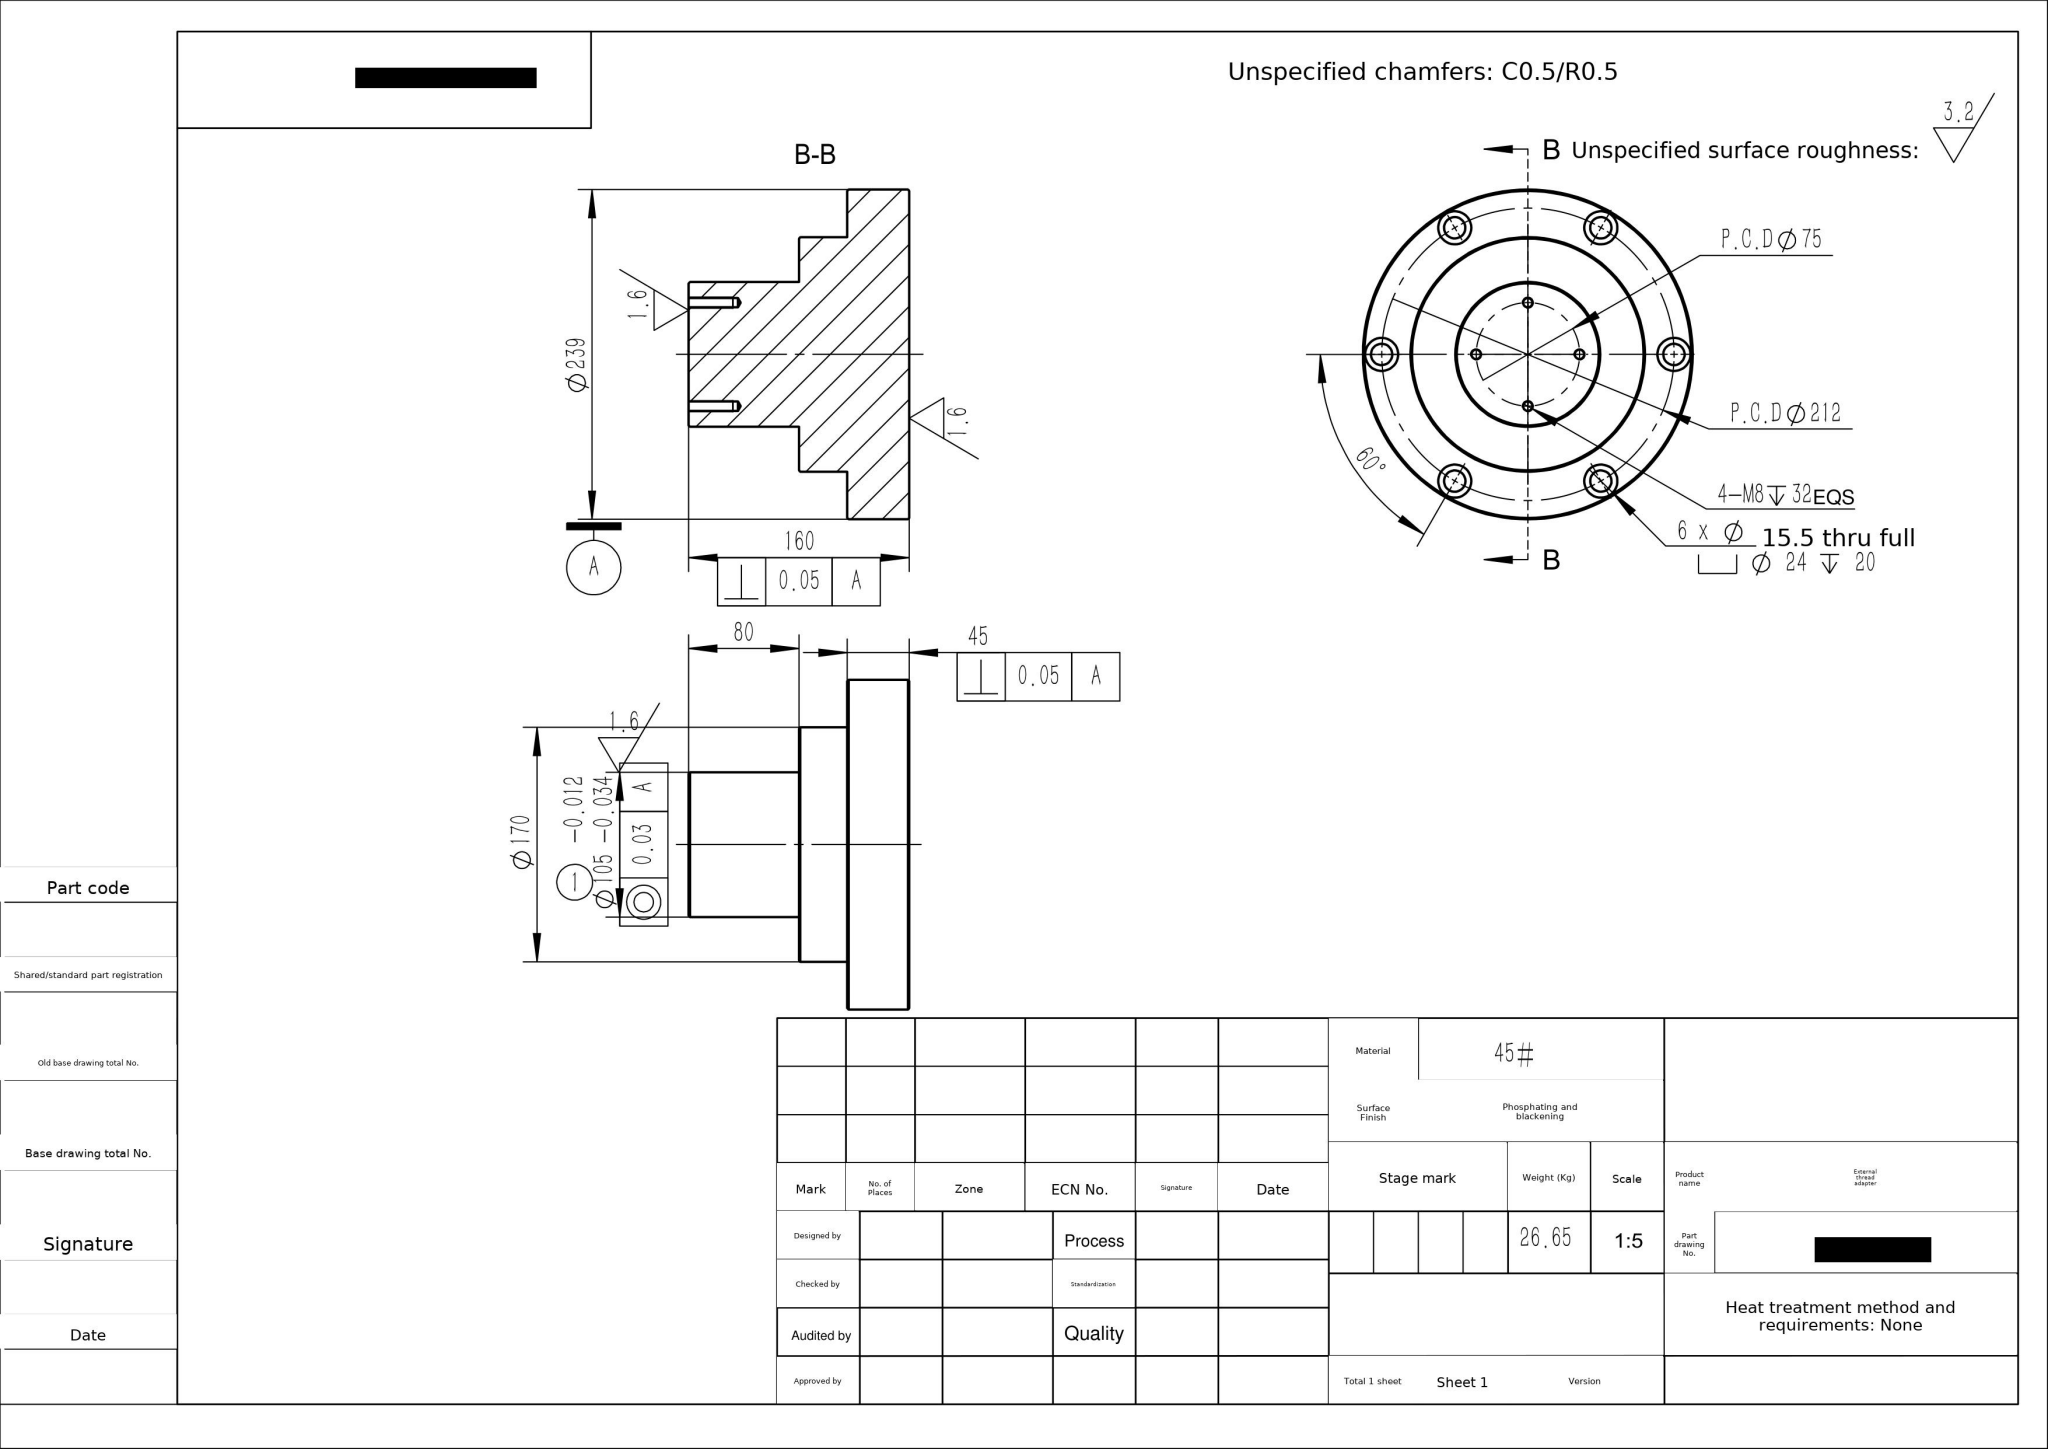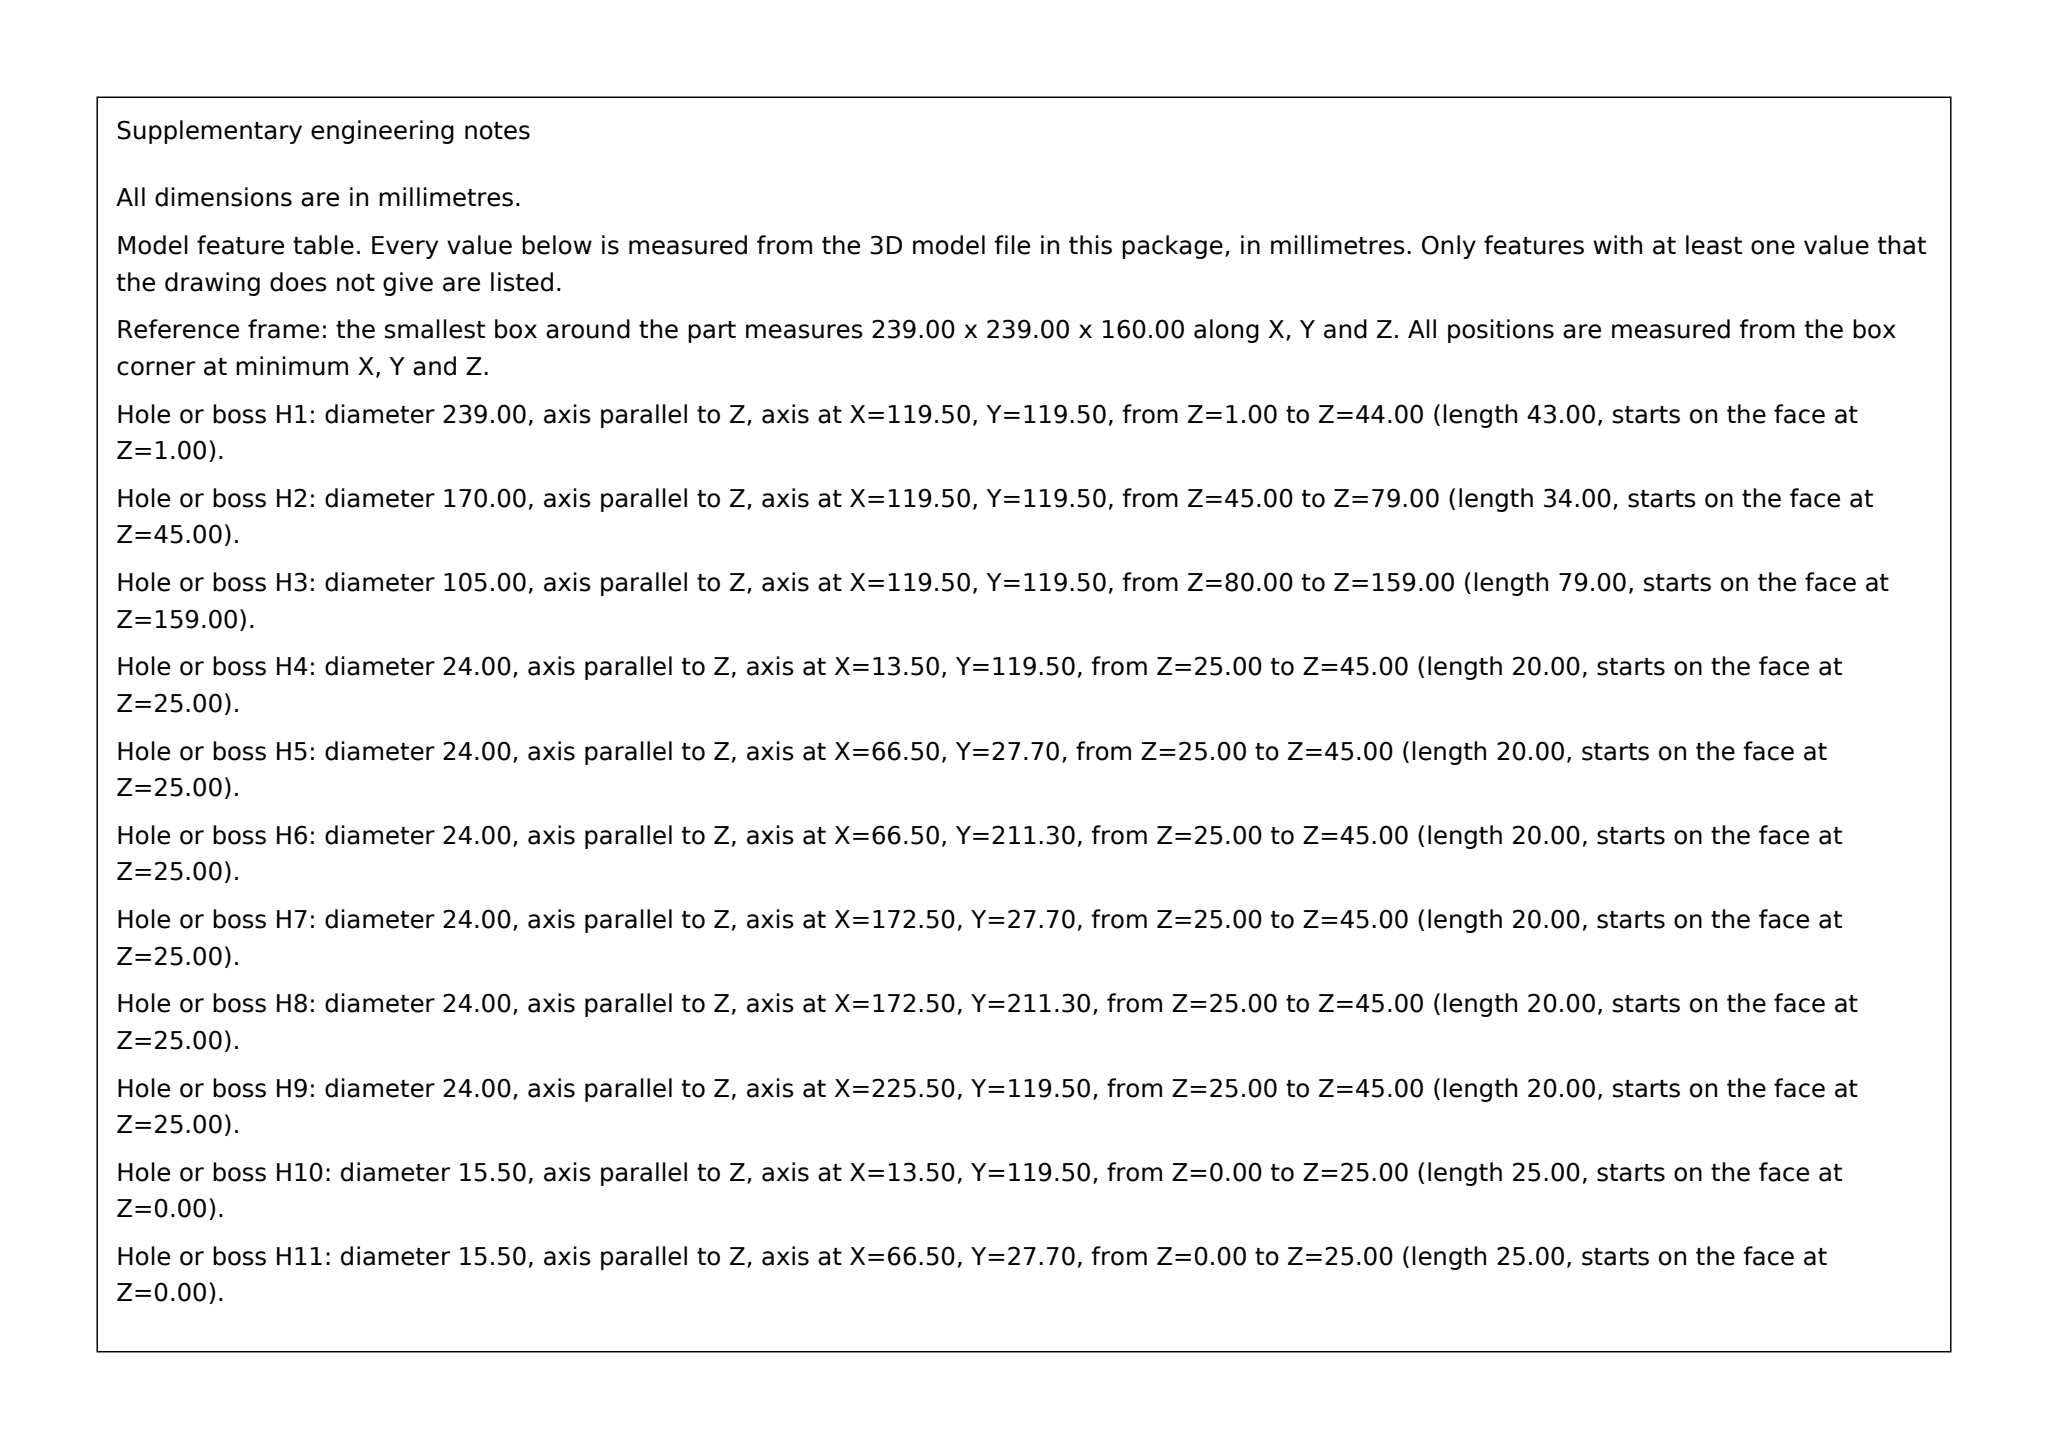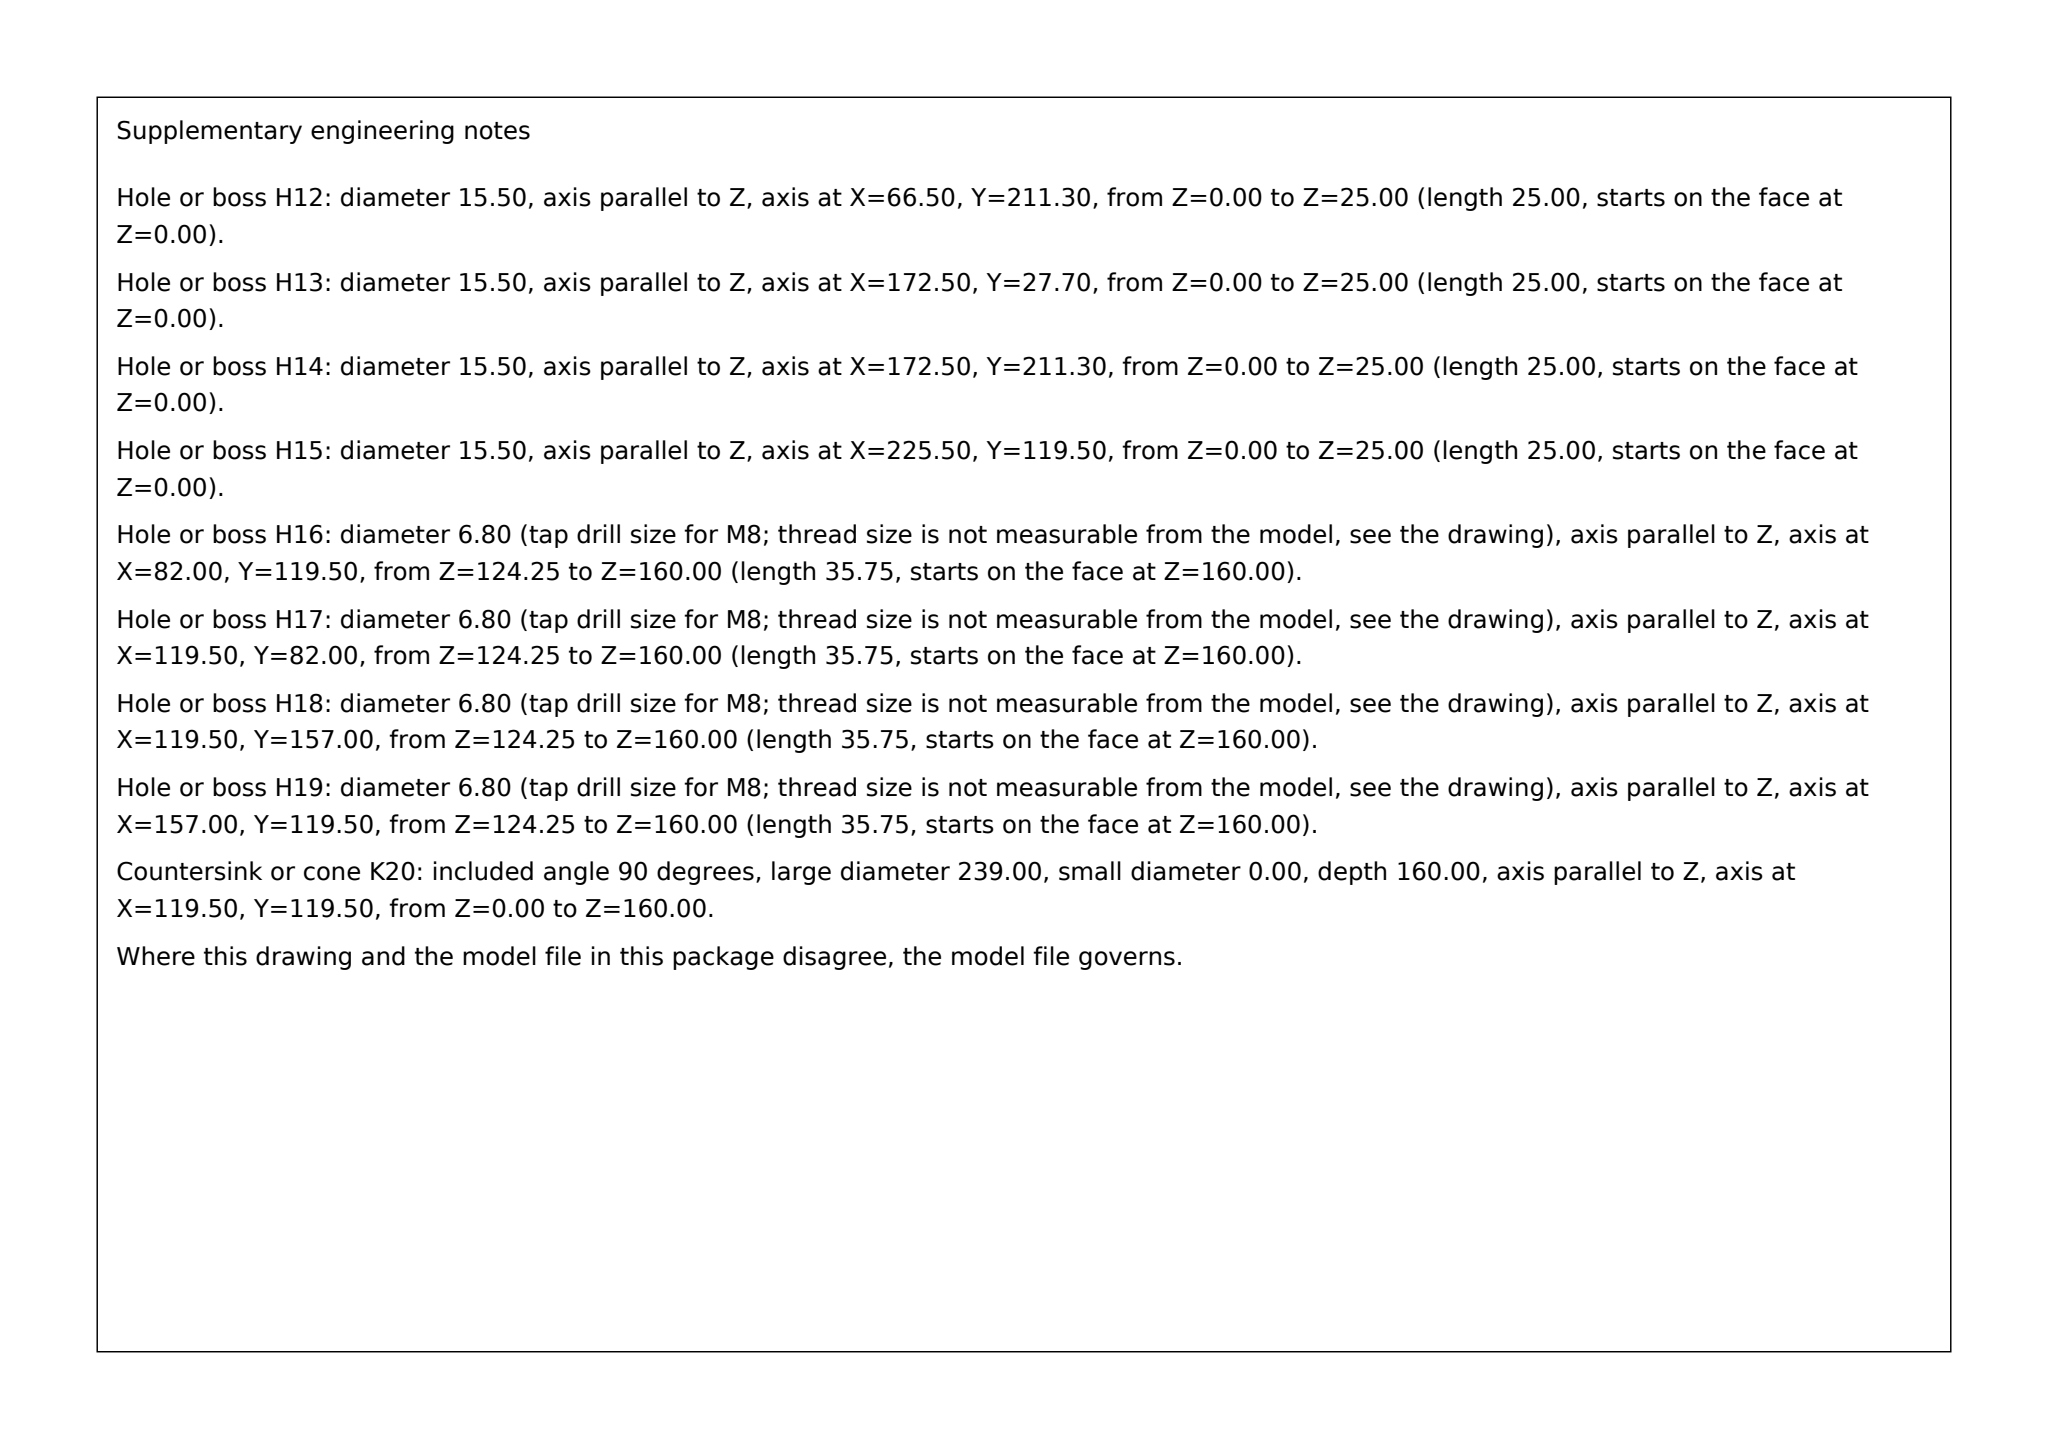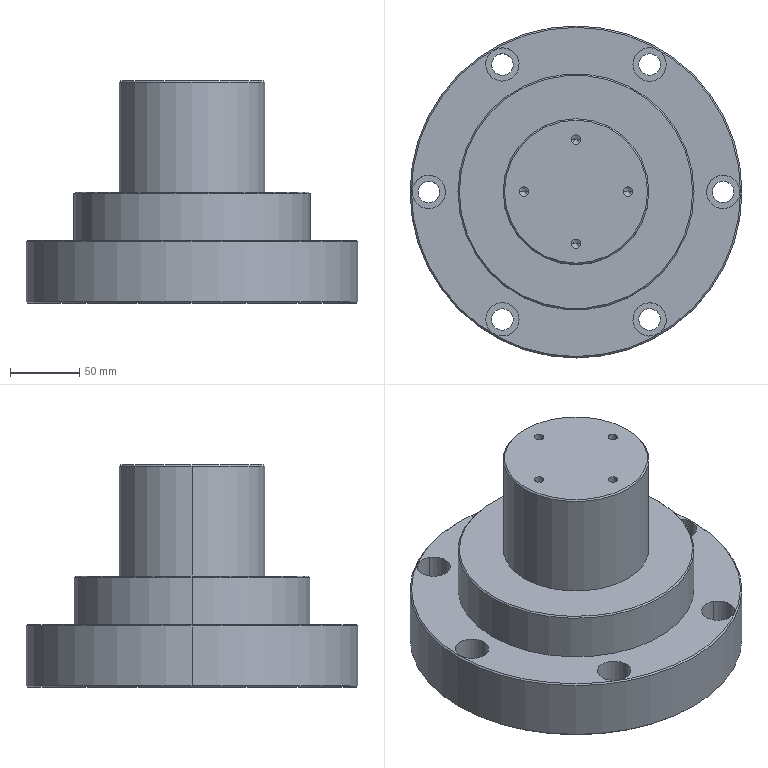Part | SolidWorks | mm | material 45# | 1 solid | 64 faces | box 239 x 239 x 160 mm | volume 3416913 mm3 | cylinder 38 | cone 16 | plane 10 | commonest cylinder face diameters 24 x12 15.5 x12 6.8 x8 105 x2 170 x2 239 x2
build123d program:
from build123d import *

# Parameters (mm, degrees)
SKETCH1_R                                         = 119.5
BOSS_EXTRUDE1_DEPTH                               = 55
SKETCH2_R                                         = 100
BOSS_EXTRUDE2_DEPTH                               = 60
SKETCH3_R                                         = 52.5
BOSS_EXTRUDE3_DEPTH                               = 115
CHAMFER1_SIZE                                     = 1
CIRPATTERN1_COUNT                                 = 4
SKETCH7_R                                         = 85
BOSS_EXTRUDE4_DEPTH                               = 35
SKETCH8_R                                         = 67.5
CUT_EXTRUDE3_DEPTH                                = 45
CHAMFER3_SIZE                                     = 1
SKETCH9_R                                         = 157.629
CUT_EXTRUDE4_DEPTH                                = 70
HOLE_SIZE_ACCORDING_TO_HEXAGON_SOCKET_D           = 15.5
HOLE_SIZE_ACCORDING_TO_HEXAGON_SOCKET_CBORE_D     = 24
HOLE_SIZE_ACCORDING_TO_HEXAGON_SOCKET_CBORE_DEPTH = 20
CIRPATTERN2_COUNT                                 = 6
CHAMFER4_SIZE                                     = 1


with BuildPart() as part:
    # Sketch1 → Boss-Extrude1 (new body)
    with BuildSketch(Plane.XY):
        Circle(SKETCH1_R)
    extrude(amount=BOSS_EXTRUDE1_DEPTH)

    # Sketch2 → Boss-Extrude2 (add)
    with BuildSketch(Plane(origin=(0, 0, 0), x_dir=(-1, 0, 0), z_dir=(0, 0, -1))):
        Circle(SKETCH2_R)
    extrude(amount=BOSS_EXTRUDE2_DEPTH)

    # Sketch3 → Boss-Extrude3 (add)
    with BuildSketch(Plane.XY.offset(55)):
        Circle(SKETCH3_R)
    extrude(amount=BOSS_EXTRUDE3_DEPTH)

    # Chamfer1
    chamfer1_edges = [part.edges().sort_by_distance(p)[0] for p in [
        (-52.5, 0, 170),
        (-119.5, 0, 0),
        (-119.5, 0, 55),
        (100, 0, -60),
    ]]
    chamfer(chamfer1_edges, length=CHAMFER1_SIZE)

    # Sketch6 → M8 Tapped Hole1 (revolve, cut)
    with BuildSketch(Plane(origin=(-37.5, 0, 170), x_dir=(0, -1, 0), z_dir=(1, 0, 0))):
        Polygon((0, 0), (0, 37.793), (3.4, 35.75), (3.4, 0), align=None)
    m8_tapped_hole1 = revolve(axis=Axis((-37.5, 0, 176.35), (0, 0, -1)), mode=Mode.SUBTRACT)

    # CirPattern1: M8 Tapped Hole1 ×4 about axis
    cirpattern1_axis = Axis((0, 0, 0), (0, 0, 1))
    for i in range(1, CIRPATTERN1_COUNT):
        add(m8_tapped_hole1.rotate(cirpattern1_axis, i * 360 / CIRPATTERN1_COUNT), mode=Mode.SUBTRACT)

    # Sketch7 → Boss-Extrude4 (add)
    with BuildSketch(Plane.XY.offset(55)):
        Circle(SKETCH7_R)
    extrude(amount=BOSS_EXTRUDE4_DEPTH)

    # Sketch8 → Cut-Extrude3 (cut)
    with BuildSketch(Plane(origin=(0, 0, -60), x_dir=(-1, 0, 0), z_dir=(0, 0, -1))):
        Circle(SKETCH8_R)
    extrude(amount=-CUT_EXTRUDE3_DEPTH, mode=Mode.SUBTRACT)

    # Chamfer3
    chamfer3_edges = [part.edges().sort_by_distance(p)[0] for p in [
        (-85, 0, 90),
    ]]
    chamfer(chamfer3_edges, length=CHAMFER3_SIZE)

    # Sketch9 → Cut-Extrude4 (cut)
    with BuildSketch(Plane(origin=(0, 0, -60), x_dir=(-1, 0, 0), z_dir=(0, 0, -1))):
        Circle(SKETCH9_R)
    extrude(amount=-CUT_EXTRUDE4_DEPTH, mode=Mode.SUBTRACT)

    # Hole Size _according to_ Hexagon Socket (through all)
    with Locations(Plane.XY.offset(55)):
        with Locations((-53, -91.799)):
            hole_size_according_to_hexagon_socket = CounterBoreHole(HOLE_SIZE_ACCORDING_TO_HEXAGON_SOCKET_D / 2, HOLE_SIZE_ACCORDING_TO_HEXAGON_SOCKET_CBORE_D / 2, HOLE_SIZE_ACCORDING_TO_HEXAGON_SOCKET_CBORE_DEPTH)

    # CirPattern2: Hole Size _according to_ Hexagon Socket ×6 about axis
    cirpattern2_axis = Axis((0, 0, 0), (0, 0, 1))
    for i in range(1, CIRPATTERN2_COUNT):
        add(hole_size_according_to_hexagon_socket.rotate(cirpattern2_axis, i * 360 / CIRPATTERN2_COUNT), mode=Mode.SUBTRACT)

    # Chamfer4
    chamfer4_edges = [part.edges().sort_by_distance(p)[0] for p in [
        (-119.5, 0, 10),
    ]]
    chamfer(chamfer4_edges, length=CHAMFER4_SIZE)


solid = part.part